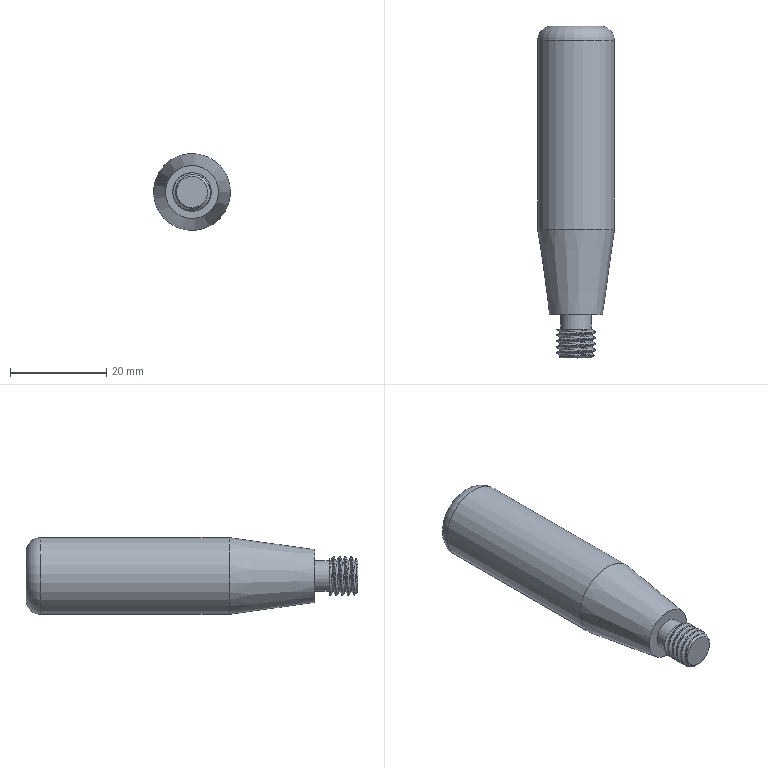Component | NX | HANDLE | 1 solid | 13 faces | volume 11319 mm3 | plane 4 | cylinder 4 | cone 2 | spline 2 | torus 1 | commonest cylinder face diameters 8 x1 6.4 x1 16 x1 6.75 x1